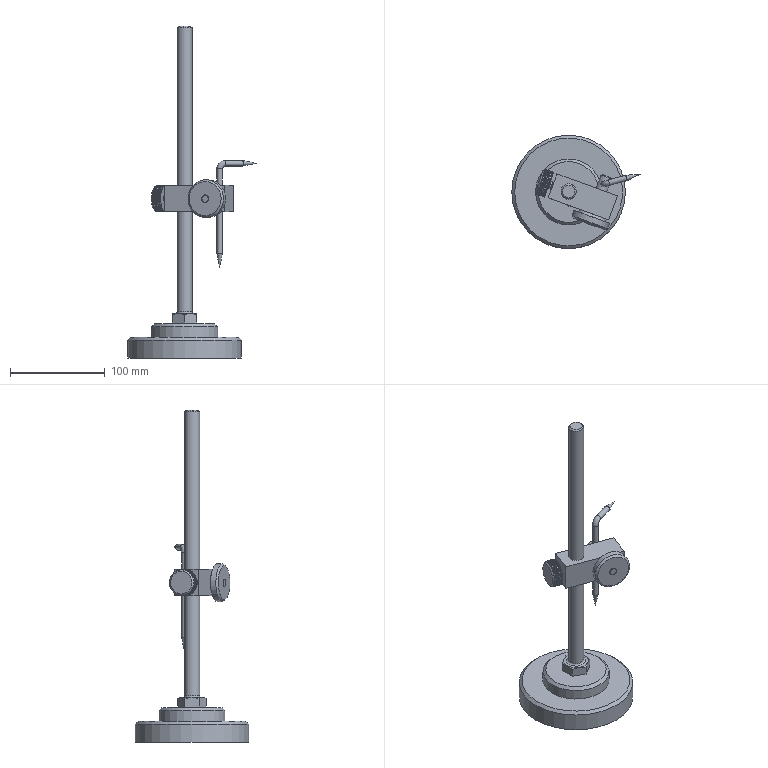Assembly | NX | mm | 7 component files | 9 solids | 426 faces | box 135.68 x 120 x 351 mm | volume 368035 mm3 | spline 213 | cylinder 155 | plane 38 | cone 16 | torus 4 | commonest cylinder face diameters 28 x100 8 x23 16 x15 6 x3 7.188 x3 12 x2 7.18 x2 14.7 x2
Bill of materials:
unnamed part 1 | 1 |  | Rectangular prismatic block with two round through-holes on perpendicular axes: one through the large top face, one through a long side face.
unnamed part 2 | 1 |  | Stepped circular disc: a wide flange with a smaller concentric raised boss, and a small central hole that looks threaded.
unnamed part 3 | 1 |  | Cylindrical pin with an externally threaded smaller-diameter end, a shoulder step, and a radial cross-hole near the plain end.
unnamed part 4 | 1 |  | Long slender cylindrical rod with a hexagonal collar near one end and a short threaded stub beyond the collar.
unnamed part 5 | 1 |  | Thin circular disc with a low concentric raised boss on one face and a central hole that looks threaded.
unnamed part 6 | 1 |  | L-shaped bent round rod with a rounded bend and conical pointed tips on both legs; one leg is much longer than the other.
unnamed part 7 | 1 |  | Screw-like part: a large cylindrical head with diamond-knurled sides, flat faces, and a smaller concentric externally threaded shank with a short neck at its base.
Mates:
1. touch align | 2 1 face | assembly face
2. touch align | 2 1 face | assembly face
3. touch align | 4 1 face | 2 1 face
4. touch align | 7 1 face | 4 1 face
5. distance | 7 1 face | 4 1 face
6. touch align | 6 1 face | 4 1 face
7. touch align | 5 1 face | 4 1 face
8. touch align | 5 1 face | 4 1 face
9. touch align | 3 1 edge | 6 1 face
10. parallel | 3 1 face | 2 1 face